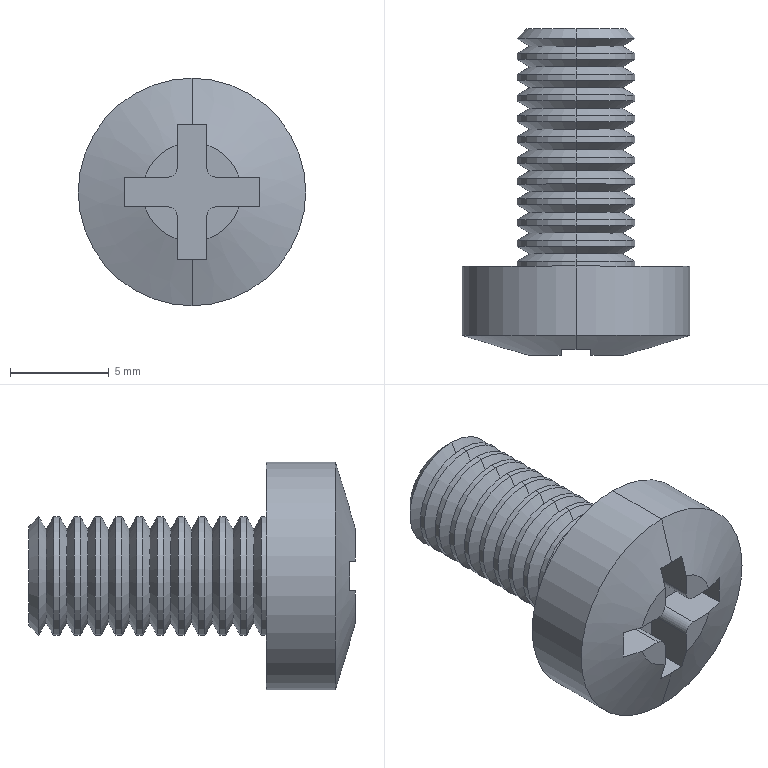Component | SolidWorks | M6PhillipsSelf-tappingScrew-1 | 1 solid | 95 faces | box 11.5 x 16.5 x 11.5 mm | volume 665 mm3 | cone 48 | cylinder 28 | plane 19 | commonest cylinder face diameters 6 x22 1 x4 11.5 x2
build123d program:
from build123d import *

# Parameters (mm, degrees)
LPATTERN1_COUNT    = 11
LPATTERN1_PITCH    = 1.05
CUT_EXTRUDE2_DEPTH = 2.5


with BuildPart() as part:
    # Sketch1 → Revolve1 (revolve)
    with BuildSketch(Plane.XY, mode=Mode.PRIVATE) as revolve1_sk:
        Polygon((-1.688, -11.759), (0.8117, -11.759), (4.062, -10.759), (4.062, -7.259), (1.312, -7.259), (1.312, 4.241), (0.8117, 4.741), (-1.688, 4.741), align=None)
    revolve(revolve1_sk.sketch.rotate(Axis((-1.688, 4.741, 0), (0, -1, 0)), 90), axis=Axis((-1.688, 4.741, 0), (0, -1, 0)))

    # Sketch2 → Cut-Revolve4 (revolve, cut)
    with BuildSketch(Plane.XY, mode=Mode.PRIVATE) as cut_revolve4_sk:
        Polygon((-4.688, 4.241), (-4.688, 3.491), (-4.039, 3.866), align=None)
    cut_revolve4 = revolve(cut_revolve4_sk.sketch.rotate(Axis((-1.688, -12.709, 0), (0, 1, 0)), 270), axis=Axis((-1.688, -12.709, 0), (0, 1, 0)), mode=Mode.SUBTRACT)

    # LPattern1: Cut-Revolve4 ×11
    with Locations(*[(0, -i * LPATTERN1_PITCH, 0) for i in range(1, LPATTERN1_COUNT)]):
        add(cut_revolve4, mode=Mode.SUBTRACT)

    # Sketch7 → Cut-Extrude2 (cut)
    with BuildSketch(Plane.XZ.offset(11.759)):
        with BuildLine():
            Line((1.73, 0.75), (-0.4383, 0.75))
            ThreePointArc((-0.4383, 0.75), (-0.7919, 0.8964), (-0.9383, 1.25))
            Line((-0.9383, 1.25), (-0.9383, 3.419))
            Line((-0.9383, 3.419), (-2.438, 3.419))
            Line((-2.438, 3.419), (-2.438, 1.25))
            ThreePointArc((-2.438, 1.25), (-2.585, 0.8964), (-2.938, 0.75))
            Line((-2.938, 0.75), (-5.107, 0.75))
            Line((-5.107, 0.75), (-5.107, -0.75))
            Line((-5.107, -0.75), (-2.938, -0.75))
            ThreePointArc((-2.938, -0.75), (-2.585, -0.8964), (-2.438, -1.25))
            Line((-2.438, -1.25), (-2.438, -3.419))
            Line((-2.438, -3.419), (-0.9383, -3.419))
            Line((-0.9383, -3.419), (-0.9383, -1.25))
            ThreePointArc((-0.9383, -1.25), (-0.7919, -0.8964), (-0.4383, -0.75))
            Line((-0.4383, -0.75), (1.73, -0.75))
            Line((1.73, -0.75), (1.73, 0.75))
        make_face()
    extrude(amount=-CUT_EXTRUDE2_DEPTH, mode=Mode.SUBTRACT)


solid = part.part

# Placed as in the assembly
solid = solid.moved(Location((524.665, 164.06, 253.01), (0, 0, 0)))